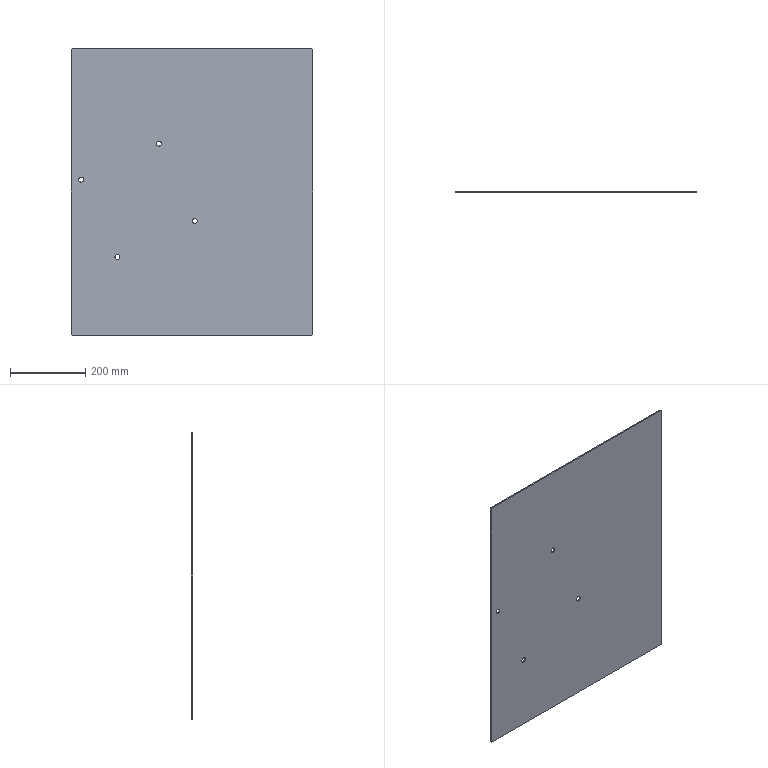Component | SolidWorks | 01-01Chassis-1_01-01-04ChassisWeldment4-1 | 1 solid | 18 faces | box 640 x 3 x 760 mm | volume 1457418 mm3 | cylinder 12 | plane 6 | commonest cylinder face diameters 13.5 x8 10 x4 | material Q235
STEP:
#1=CARTESIAN_POINT('',(-3.474,1.575,4.786));
#2=VERTEX_POINT('',#1);
#3=CARTESIAN_POINT('',(-3.474,1.575,5.317));
#4=VERTEX_POINT('',#3);
#5=CARTESIAN_POINT('',(-3.474,1.575,5.052));
#6=DIRECTION('',(0.,1.,0.));
#7=DIRECTION('',(0.,0.,1.));
#8=AXIS2_PLACEMENT_3D('',#5,#6,#7);
#9=CIRCLE('',#8,0.2657);
#10=EDGE_CURVE('',#2,#4,#9,.T.);
#11=ORIENTED_EDGE('',*,*,#10,.F.);
#12=CARTESIAN_POINT('',(-3.474,1.693,4.786));
#13=VERTEX_POINT('',#12);
#14=CARTESIAN_POINT('',(-3.474,1.575,4.786));
#15=DIRECTION('',(0.,1.,0.));
#16=VECTOR('',#15,39.37);
#17=LINE('',#14,#16);
#18=EDGE_CURVE('',#2,#13,#17,.T.);
#19=ORIENTED_EDGE('',*,*,#18,.T.);
#20=CARTESIAN_POINT('',(-3.474,1.693,5.317));
#21=VERTEX_POINT('',#20);
#22=CARTESIAN_POINT('',(-3.474,1.693,5.052));
#23=DIRECTION('',(0.,1.,0.));
#24=DIRECTION('',(0.,0.,1.));
#25=AXIS2_PLACEMENT_3D('',#22,#23,#24);
#26=CIRCLE('',#25,0.2657);
#27=EDGE_CURVE('',#13,#21,#26,.T.);
#28=ORIENTED_EDGE('',*,*,#27,.T.);
#29=CARTESIAN_POINT('',(-3.474,1.575,5.317));
#30=DIRECTION('',(0.,1.,0.));
#31=VECTOR('',#30,39.37);
#32=LINE('',#29,#31);
#33=EDGE_CURVE('',#4,#21,#32,.T.);
#34=ORIENTED_EDGE('',*,*,#33,.F.);
#35=EDGE_LOOP('',(#11,#19,#28,#34));
#36=FACE_OUTER_BOUND('',#35,.T.);
#37=CARTESIAN_POINT('',(-3.474,1.575,5.052));
#38=DIRECTION('',(0.,1.,0.));
#39=DIRECTION('',(0.,0.,1.));
#40=AXIS2_PLACEMENT_3D('',#37,#38,#39);
#41=CYLINDRICAL_SURFACE('',#40,0.2657);
#42=ADVANCED_FACE('',(#36),#41,.F.);
#43=CARTESIAN_POINT('',(0.291,1.575,-3.288));
#44=VERTEX_POINT('',#43);
#45=CARTESIAN_POINT('',(0.291,1.575,-2.756));
#46=VERTEX_POINT('',#45);
#47=CARTESIAN_POINT('',(0.291,1.575,-3.022));
#48=DIRECTION('',(0.,1.,0.));
#49=DIRECTION('',(0.,0.,1.));
#50=AXIS2_PLACEMENT_3D('',#47,#48,#49);
#51=CIRCLE('',#50,0.2657);
#52=EDGE_CURVE('',#44,#46,#51,.T.);
#53=ORIENTED_EDGE('',*,*,#52,.F.);
#54=CARTESIAN_POINT('',(0.291,1.693,-3.288));
#55=VERTEX_POINT('',#54);
#56=CARTESIAN_POINT('',(0.291,1.575,-3.288));
#57=DIRECTION('',(0.,1.,0.));
#58=VECTOR('',#57,39.37);
#59=LINE('',#56,#58);
#60=EDGE_CURVE('',#44,#55,#59,.T.);
#61=ORIENTED_EDGE('',*,*,#60,.T.);
#62=CARTESIAN_POINT('',(0.291,1.693,-2.756));
#63=VERTEX_POINT('',#62);
#64=CARTESIAN_POINT('',(0.291,1.693,-3.022));
#65=DIRECTION('',(0.,1.,0.));
#66=DIRECTION('',(0.,0.,1.));
#67=AXIS2_PLACEMENT_3D('',#64,#65,#66);
#68=CIRCLE('',#67,0.2657);
#69=EDGE_CURVE('',#55,#63,#68,.T.);
#70=ORIENTED_EDGE('',*,*,#69,.T.);
#71=CARTESIAN_POINT('',(0.291,1.575,-2.756));
#72=DIRECTION('',(0.,1.,0.));
#73=VECTOR('',#72,39.37);
#74=LINE('',#71,#73);
#75=EDGE_CURVE('',#46,#63,#74,.T.);
#76=ORIENTED_EDGE('',*,*,#75,.F.);
#77=EDGE_LOOP('',(#53,#61,#70,#76));
#78=FACE_OUTER_BOUND('',#77,.T.);
#79=CARTESIAN_POINT('',(0.291,1.575,-3.022));
#80=DIRECTION('',(0.,1.,0.));
#81=DIRECTION('',(0.,0.,1.));
#82=AXIS2_PLACEMENT_3D('',#79,#80,#81);
#83=CYLINDRICAL_SURFACE('',#82,0.2657);
#84=ADVANCED_FACE('',(#78),#83,.F.);
#85=CARTESIAN_POINT('',(-7.783,1.575,-7.053));
#86=VERTEX_POINT('',#85);
#87=CARTESIAN_POINT('',(-7.783,1.575,-6.521));
#88=VERTEX_POINT('',#87);
#89=CARTESIAN_POINT('',(-7.783,1.575,-6.787));
#90=DIRECTION('',(0.,1.,0.));
#91=DIRECTION('',(0.,0.,1.));
#92=AXIS2_PLACEMENT_3D('',#89,#90,#91);
#93=CIRCLE('',#92,0.2657);
#94=EDGE_CURVE('',#86,#88,#93,.T.);
#95=ORIENTED_EDGE('',*,*,#94,.F.);
#96=CARTESIAN_POINT('',(-7.783,1.693,-7.053));
#97=VERTEX_POINT('',#96);
#98=CARTESIAN_POINT('',(-7.783,1.575,-7.053));
#99=DIRECTION('',(0.,1.,0.));
#100=VECTOR('',#99,39.37);
#101=LINE('',#98,#100);
#102=EDGE_CURVE('',#86,#97,#101,.T.);
#103=ORIENTED_EDGE('',*,*,#102,.T.);
#104=CARTESIAN_POINT('',(-7.783,1.693,-6.521));
#105=VERTEX_POINT('',#104);
#106=CARTESIAN_POINT('',(-7.783,1.693,-6.787));
#107=DIRECTION('',(0.,1.,0.));
#108=DIRECTION('',(0.,0.,1.));
#109=AXIS2_PLACEMENT_3D('',#106,#107,#108);
#110=CIRCLE('',#109,0.2657);
#111=EDGE_CURVE('',#97,#105,#110,.T.);
#112=ORIENTED_EDGE('',*,*,#111,.T.);
#113=CARTESIAN_POINT('',(-7.783,1.575,-6.521));
#114=DIRECTION('',(0.,1.,0.));
#115=VECTOR('',#114,39.37);
#116=LINE('',#113,#115);
#117=EDGE_CURVE('',#88,#105,#116,.T.);
#118=ORIENTED_EDGE('',*,*,#117,.F.);
#119=EDGE_LOOP('',(#95,#103,#112,#118));
#120=FACE_OUTER_BOUND('',#119,.T.);
#121=CARTESIAN_POINT('',(-7.783,1.575,-6.787));
#122=DIRECTION('',(0.,1.,0.));
#123=DIRECTION('',(0.,0.,1.));
#124=AXIS2_PLACEMENT_3D('',#121,#122,#123);
#125=CYLINDRICAL_SURFACE('',#124,0.2657);
#126=ADVANCED_FACE('',(#120),#125,.F.);
#127=CARTESIAN_POINT('',(-11.548,1.575,1.021));
#128=VERTEX_POINT('',#127);
#129=CARTESIAN_POINT('',(-11.548,1.575,1.553));
#130=VERTEX_POINT('',#129);
#131=CARTESIAN_POINT('',(-11.548,1.575,1.287));
#132=DIRECTION('',(0.,1.,0.));
#133=DIRECTION('',(0.,0.,1.));
#134=AXIS2_PLACEMENT_3D('',#131,#132,#133);
#135=CIRCLE('',#134,0.2657);
#136=EDGE_CURVE('',#128,#130,#135,.T.);
#137=ORIENTED_EDGE('',*,*,#136,.F.);
#138=CARTESIAN_POINT('',(-11.548,1.693,1.021));
#139=VERTEX_POINT('',#138);
#140=CARTESIAN_POINT('',(-11.548,1.575,1.021));
#141=DIRECTION('',(0.,1.,0.));
#142=VECTOR('',#141,39.37);
#143=LINE('',#140,#142);
#144=EDGE_CURVE('',#128,#139,#143,.T.);
#145=ORIENTED_EDGE('',*,*,#144,.T.);
#146=CARTESIAN_POINT('',(-11.548,1.693,1.553));
#147=VERTEX_POINT('',#146);
#148=CARTESIAN_POINT('',(-11.548,1.693,1.287));
#149=DIRECTION('',(0.,1.,0.));
#150=DIRECTION('',(0.,0.,1.));
#151=AXIS2_PLACEMENT_3D('',#148,#149,#150);
#152=CIRCLE('',#151,0.2657);
#153=EDGE_CURVE('',#139,#147,#152,.T.);
#154=ORIENTED_EDGE('',*,*,#153,.T.);
#155=CARTESIAN_POINT('',(-11.548,1.575,1.553));
#156=DIRECTION('',(0.,1.,0.));
#157=VECTOR('',#156,39.37);
#158=LINE('',#155,#157);
#159=EDGE_CURVE('',#130,#147,#158,.T.);
#160=ORIENTED_EDGE('',*,*,#159,.F.);
#161=EDGE_LOOP('',(#137,#145,#154,#160));
#162=FACE_OUTER_BOUND('',#161,.T.);
#163=CARTESIAN_POINT('',(-11.548,1.575,1.287));
#164=DIRECTION('',(0.,1.,0.));
#165=DIRECTION('',(0.,0.,1.));
#166=AXIS2_PLACEMENT_3D('',#163,#164,#165);
#167=CYLINDRICAL_SURFACE('',#166,0.2657);
#168=ADVANCED_FACE('',(#162),#167,.F.);
#169=CARTESIAN_POINT('',(-12.598,1.693,14.764));
#170=VERTEX_POINT('',#169);
#171=CARTESIAN_POINT('',(-12.402,1.693,14.961));
#172=VERTEX_POINT('',#171);
#173=CARTESIAN_POINT('',(-12.402,1.693,14.764));
#174=DIRECTION('',(0.,1.,0.));
#175=DIRECTION('',(0.,0.,-1.));
#176=AXIS2_PLACEMENT_3D('',#173,#174,#175);
#177=CIRCLE('',#176,0.1969);
#178=EDGE_CURVE('',#170,#172,#177,.T.);
#179=ORIENTED_EDGE('',*,*,#178,.F.);
#180=CARTESIAN_POINT('',(-12.598,1.575,14.764));
#181=VERTEX_POINT('',#180);
#182=CARTESIAN_POINT('',(-12.598,1.575,14.764));
#183=DIRECTION('',(0.,1.,0.));
#184=VECTOR('',#183,39.37);
#185=LINE('',#182,#184);
#186=EDGE_CURVE('',#181,#170,#185,.T.);
#187=ORIENTED_EDGE('',*,*,#186,.F.);
#188=CARTESIAN_POINT('',(-12.402,1.575,14.961));
#189=VERTEX_POINT('',#188);
#190=CARTESIAN_POINT('',(-12.402,1.575,14.764));
#191=DIRECTION('',(0.,1.,0.));
#192=DIRECTION('',(0.,0.,-1.));
#193=AXIS2_PLACEMENT_3D('',#190,#191,#192);
#194=CIRCLE('',#193,0.1969);
#195=EDGE_CURVE('',#181,#189,#194,.T.);
#196=ORIENTED_EDGE('',*,*,#195,.T.);
#197=CARTESIAN_POINT('',(-12.402,1.575,14.961));
#198=DIRECTION('',(0.,1.,0.));
#199=VECTOR('',#198,39.37);
#200=LINE('',#197,#199);
#201=EDGE_CURVE('',#189,#172,#200,.T.);
#202=ORIENTED_EDGE('',*,*,#201,.T.);
#203=EDGE_LOOP('',(#179,#187,#196,#202));
#204=FACE_OUTER_BOUND('',#203,.T.);
#205=CARTESIAN_POINT('',(-12.402,1.575,14.764));
#206=DIRECTION('',(0.,1.,0.));
#207=DIRECTION('',(0.,0.,1.));
#208=AXIS2_PLACEMENT_3D('',#205,#206,#207);
#209=CYLINDRICAL_SURFACE('',#208,0.1969);
#210=ADVANCED_FACE('',(#204),#209,.T.);
#211=CARTESIAN_POINT('',(-12.598,1.693,-14.764));
#212=VERTEX_POINT('',#211);
#213=CARTESIAN_POINT('',(-12.598,1.693,14.764));
#214=DIRECTION('',(0.,0.,1.));
#215=VECTOR('',#214,39.37);
#216=LINE('',#213,#215);
#217=EDGE_CURVE('',#212,#170,#216,.T.);
#218=ORIENTED_EDGE('',*,*,#217,.F.);
#219=CARTESIAN_POINT('',(-12.598,1.575,-14.764));
#220=VERTEX_POINT('',#219);
#221=CARTESIAN_POINT('',(-12.598,1.575,-14.764));
#222=DIRECTION('',(0.,1.,0.));
#223=VECTOR('',#222,39.37);
#224=LINE('',#221,#223);
#225=EDGE_CURVE('',#220,#212,#224,.T.);
#226=ORIENTED_EDGE('',*,*,#225,.F.);
#227=CARTESIAN_POINT('',(-12.598,1.575,14.764));
#228=DIRECTION('',(0.,0.,1.));
#229=VECTOR('',#228,39.37);
#230=LINE('',#227,#229);
#231=EDGE_CURVE('',#220,#181,#230,.T.);
#232=ORIENTED_EDGE('',*,*,#231,.T.);
#233=ORIENTED_EDGE('',*,*,#186,.T.);
#234=EDGE_LOOP('',(#218,#226,#232,#233));
#235=FACE_OUTER_BOUND('',#234,.T.);
#236=CARTESIAN_POINT('',(-12.598,1.575,14.764));
#237=DIRECTION('',(-1.,0.,0.));
#238=DIRECTION('',(0.,0.,1.));
#239=AXIS2_PLACEMENT_3D('',#236,#237,#238);
#240=PLANE('',#239);
#241=ADVANCED_FACE('',(#235),#240,.T.);
#242=CARTESIAN_POINT('',(-12.402,1.693,-14.961));
#243=VERTEX_POINT('',#242);
#244=CARTESIAN_POINT('',(-12.402,1.693,-14.764));
#245=DIRECTION('',(0.,1.,0.));
#246=DIRECTION('',(0.,0.,1.));
#247=AXIS2_PLACEMENT_3D('',#244,#245,#246);
#248=CIRCLE('',#247,0.1969);
#249=EDGE_CURVE('',#243,#212,#248,.T.);
#250=ORIENTED_EDGE('',*,*,#249,.F.);
#251=CARTESIAN_POINT('',(-12.402,1.575,-14.961));
#252=VERTEX_POINT('',#251);
#253=CARTESIAN_POINT('',(-12.402,1.575,-14.961));
#254=DIRECTION('',(0.,1.,0.));
#255=VECTOR('',#254,39.37);
#256=LINE('',#253,#255);
#257=EDGE_CURVE('',#252,#243,#256,.T.);
#258=ORIENTED_EDGE('',*,*,#257,.F.);
#259=CARTESIAN_POINT('',(-12.402,1.575,-14.764));
#260=DIRECTION('',(0.,1.,0.));
#261=DIRECTION('',(0.,0.,1.));
#262=AXIS2_PLACEMENT_3D('',#259,#260,#261);
#263=CIRCLE('',#262,0.1969);
#264=EDGE_CURVE('',#252,#220,#263,.T.);
#265=ORIENTED_EDGE('',*,*,#264,.T.);
#266=ORIENTED_EDGE('',*,*,#225,.T.);
#267=EDGE_LOOP('',(#250,#258,#265,#266));
#268=FACE_OUTER_BOUND('',#267,.T.);
#269=CARTESIAN_POINT('',(-12.402,1.575,-14.764));
#270=DIRECTION('',(0.,1.,0.));
#271=DIRECTION('',(0.,0.,1.));
#272=AXIS2_PLACEMENT_3D('',#269,#270,#271);
#273=CYLINDRICAL_SURFACE('',#272,0.1969);
#274=ADVANCED_FACE('',(#268),#273,.T.);
#275=CARTESIAN_POINT('',(12.402,1.693,-14.961));
#276=VERTEX_POINT('',#275);
#277=CARTESIAN_POINT('',(12.402,1.693,-14.961));
#278=DIRECTION('',(-1.,0.,0.));
#279=VECTOR('',#278,39.37);
#280=LINE('',#277,#279);
#281=EDGE_CURVE('',#276,#243,#280,.T.);
#282=ORIENTED_EDGE('',*,*,#281,.F.);
#283=CARTESIAN_POINT('',(12.402,1.575,-14.961));
#284=VERTEX_POINT('',#283);
#285=CARTESIAN_POINT('',(12.402,1.575,-14.961));
#286=DIRECTION('',(0.,1.,0.));
#287=VECTOR('',#286,39.37);
#288=LINE('',#285,#287);
#289=EDGE_CURVE('',#284,#276,#288,.T.);
#290=ORIENTED_EDGE('',*,*,#289,.F.);
#291=CARTESIAN_POINT('',(12.402,1.575,-14.961));
#292=DIRECTION('',(-1.,0.,0.));
#293=VECTOR('',#292,39.37);
#294=LINE('',#291,#293);
#295=EDGE_CURVE('',#284,#252,#294,.T.);
#296=ORIENTED_EDGE('',*,*,#295,.T.);
#297=ORIENTED_EDGE('',*,*,#257,.T.);
#298=EDGE_LOOP('',(#282,#290,#296,#297));
#299=FACE_OUTER_BOUND('',#298,.T.);
#300=CARTESIAN_POINT('',(12.402,1.575,-14.961));
#301=DIRECTION('',(-0.,0.,-1.));
#302=DIRECTION('',(-1.,0.,0.));
#303=AXIS2_PLACEMENT_3D('',#300,#301,#302);
#304=PLANE('',#303);
#305=ADVANCED_FACE('',(#299),#304,.T.);
#306=CARTESIAN_POINT('',(12.598,1.693,-14.764));
#307=VERTEX_POINT('',#306);
#308=CARTESIAN_POINT('',(12.402,1.693,-14.764));
#309=DIRECTION('',(0.,1.,0.));
#310=DIRECTION('',(0.,0.,1.));
#311=AXIS2_PLACEMENT_3D('',#308,#309,#310);
#312=CIRCLE('',#311,0.1969);
#313=EDGE_CURVE('',#307,#276,#312,.T.);
#314=ORIENTED_EDGE('',*,*,#313,.F.);
#315=CARTESIAN_POINT('',(12.598,1.575,-14.764));
#316=VERTEX_POINT('',#315);
#317=CARTESIAN_POINT('',(12.598,1.575,-14.764));
#318=DIRECTION('',(0.,1.,0.));
#319=VECTOR('',#318,39.37);
#320=LINE('',#317,#319);
#321=EDGE_CURVE('',#316,#307,#320,.T.);
#322=ORIENTED_EDGE('',*,*,#321,.F.);
#323=CARTESIAN_POINT('',(12.402,1.575,-14.764));
#324=DIRECTION('',(0.,1.,0.));
#325=DIRECTION('',(0.,0.,1.));
#326=AXIS2_PLACEMENT_3D('',#323,#324,#325);
#327=CIRCLE('',#326,0.1969);
#328=EDGE_CURVE('',#316,#284,#327,.T.);
#329=ORIENTED_EDGE('',*,*,#328,.T.);
#330=ORIENTED_EDGE('',*,*,#289,.T.);
#331=EDGE_LOOP('',(#314,#322,#329,#330));
#332=FACE_OUTER_BOUND('',#331,.T.);
#333=CARTESIAN_POINT('',(12.402,1.575,-14.764));
#334=DIRECTION('',(0.,1.,0.));
#335=DIRECTION('',(0.,0.,1.));
#336=AXIS2_PLACEMENT_3D('',#333,#334,#335);
#337=CYLINDRICAL_SURFACE('',#336,0.1969);
#338=ADVANCED_FACE('',(#332),#337,.T.);
#339=CARTESIAN_POINT('',(12.598,1.693,14.764));
#340=VERTEX_POINT('',#339);
#341=CARTESIAN_POINT('',(12.598,1.693,14.764));
#342=DIRECTION('',(0.,0.,-1.));
#343=VECTOR('',#342,39.37);
#344=LINE('',#341,#343);
#345=EDGE_CURVE('',#340,#307,#344,.T.);
#346=ORIENTED_EDGE('',*,*,#345,.F.);
#347=CARTESIAN_POINT('',(12.598,1.575,14.764));
#348=VERTEX_POINT('',#347);
#349=CARTESIAN_POINT('',(12.598,1.575,14.764));
#350=DIRECTION('',(0.,1.,0.));
#351=VECTOR('',#350,39.37);
#352=LINE('',#349,#351);
#353=EDGE_CURVE('',#348,#340,#352,.T.);
#354=ORIENTED_EDGE('',*,*,#353,.F.);
#355=CARTESIAN_POINT('',(12.598,1.575,14.764));
#356=DIRECTION('',(0.,0.,-1.));
#357=VECTOR('',#356,39.37);
#358=LINE('',#355,#357);
#359=EDGE_CURVE('',#348,#316,#358,.T.);
#360=ORIENTED_EDGE('',*,*,#359,.T.);
#361=ORIENTED_EDGE('',*,*,#321,.T.);
#362=EDGE_LOOP('',(#346,#354,#360,#361));
#363=FACE_OUTER_BOUND('',#362,.T.);
#364=CARTESIAN_POINT('',(12.598,1.575,14.764));
#365=DIRECTION('',(1.,0.,0.));
#366=DIRECTION('',(0.,0.,-1.));
#367=AXIS2_PLACEMENT_3D('',#364,#365,#366);
#368=PLANE('',#367);
#369=ADVANCED_FACE('',(#363),#368,.T.);
#370=CARTESIAN_POINT('',(12.402,1.693,14.961));
#371=VERTEX_POINT('',#370);
#372=CARTESIAN_POINT('',(12.402,1.693,14.764));
#373=DIRECTION('',(0.,1.,0.));
#374=DIRECTION('',(0.,0.,1.));
#375=AXIS2_PLACEMENT_3D('',#372,#373,#374);
#376=CIRCLE('',#375,0.1969);
#377=EDGE_CURVE('',#371,#340,#376,.T.);
#378=ORIENTED_EDGE('',*,*,#377,.F.);
#379=CARTESIAN_POINT('',(12.402,1.575,14.961));
#380=VERTEX_POINT('',#379);
#381=CARTESIAN_POINT('',(12.402,1.575,14.961));
#382=DIRECTION('',(0.,1.,0.));
#383=VECTOR('',#382,39.37);
#384=LINE('',#381,#383);
#385=EDGE_CURVE('',#380,#371,#384,.T.);
#386=ORIENTED_EDGE('',*,*,#385,.F.);
#387=CARTESIAN_POINT('',(12.402,1.575,14.764));
#388=DIRECTION('',(0.,1.,0.));
#389=DIRECTION('',(0.,0.,1.));
#390=AXIS2_PLACEMENT_3D('',#387,#388,#389);
#391=CIRCLE('',#390,0.1969);
#392=EDGE_CURVE('',#380,#348,#391,.T.);
#393=ORIENTED_EDGE('',*,*,#392,.T.);
#394=ORIENTED_EDGE('',*,*,#353,.T.);
#395=EDGE_LOOP('',(#378,#386,#393,#394));
#396=FACE_OUTER_BOUND('',#395,.T.);
#397=CARTESIAN_POINT('',(12.402,1.575,14.764));
#398=DIRECTION('',(0.,1.,0.));
#399=DIRECTION('',(0.,0.,1.));
#400=AXIS2_PLACEMENT_3D('',#397,#398,#399);
#401=CYLINDRICAL_SURFACE('',#400,0.1969);
#402=ADVANCED_FACE('',(#396),#401,.T.);
#403=CARTESIAN_POINT('',(12.402,1.693,14.961));
#404=DIRECTION('',(1.,0.,-0.));
#405=VECTOR('',#404,39.37);
#406=LINE('',#403,#405);
#407=EDGE_CURVE('',#172,#371,#406,.T.);
#408=ORIENTED_EDGE('',*,*,#407,.F.);
#409=ORIENTED_EDGE('',*,*,#201,.F.);
#410=CARTESIAN_POINT('',(12.402,1.575,14.961));
#411=DIRECTION('',(1.,0.,-0.));
#412=VECTOR('',#411,39.37);
#413=LINE('',#410,#412);
#414=EDGE_CURVE('',#189,#380,#413,.T.);
#415=ORIENTED_EDGE('',*,*,#414,.T.);
#416=ORIENTED_EDGE('',*,*,#385,.T.);
#417=EDGE_LOOP('',(#408,#409,#415,#416));
#418=FACE_OUTER_BOUND('',#417,.T.);
#419=CARTESIAN_POINT('',(12.402,1.575,14.961));
#420=DIRECTION('',(0.,0.,1.));
#421=DIRECTION('',(1.,0.,-0.));
#422=AXIS2_PLACEMENT_3D('',#419,#420,#421);
#423=PLANE('',#422);
#424=ADVANCED_FACE('',(#418),#423,.T.);
#425=CARTESIAN_POINT('',(-3.474,1.575,5.052));
#426=DIRECTION('',(0.,1.,0.));
#427=DIRECTION('',(0.,0.,1.));
#428=AXIS2_PLACEMENT_3D('',#425,#426,#427);
#429=CIRCLE('',#428,0.2657);
#430=EDGE_CURVE('',#4,#2,#429,.T.);
#431=ORIENTED_EDGE('',*,*,#430,.T.);
#432=ORIENTED_EDGE('',*,*,#10,.T.);
#433=EDGE_LOOP('',(#431,#432));
#434=FACE_BOUND('',#433,.T.);
#435=CARTESIAN_POINT('',(0.291,1.575,-3.022));
#436=DIRECTION('',(0.,1.,0.));
#437=DIRECTION('',(0.,0.,1.));
#438=AXIS2_PLACEMENT_3D('',#435,#436,#437);
#439=CIRCLE('',#438,0.2657);
#440=EDGE_CURVE('',#46,#44,#439,.T.);
#441=ORIENTED_EDGE('',*,*,#440,.T.);
#442=ORIENTED_EDGE('',*,*,#52,.T.);
#443=EDGE_LOOP('',(#441,#442));
#444=FACE_BOUND('',#443,.T.);
#445=CARTESIAN_POINT('',(-7.783,1.575,-6.787));
#446=DIRECTION('',(0.,1.,0.));
#447=DIRECTION('',(0.,0.,1.));
#448=AXIS2_PLACEMENT_3D('',#445,#446,#447);
#449=CIRCLE('',#448,0.2657);
#450=EDGE_CURVE('',#88,#86,#449,.T.);
#451=ORIENTED_EDGE('',*,*,#450,.T.);
#452=ORIENTED_EDGE('',*,*,#94,.T.);
#453=EDGE_LOOP('',(#451,#452));
#454=FACE_BOUND('',#453,.T.);
#455=CARTESIAN_POINT('',(-11.548,1.575,1.287));
#456=DIRECTION('',(0.,1.,0.));
#457=DIRECTION('',(0.,0.,1.));
#458=AXIS2_PLACEMENT_3D('',#455,#456,#457);
#459=CIRCLE('',#458,0.2657);
#460=EDGE_CURVE('',#130,#128,#459,.T.);
#461=ORIENTED_EDGE('',*,*,#460,.T.);
#462=ORIENTED_EDGE('',*,*,#136,.T.);
#463=EDGE_LOOP('',(#461,#462));
#464=FACE_BOUND('',#463,.T.);
#465=ORIENTED_EDGE('',*,*,#195,.F.);
#466=ORIENTED_EDGE('',*,*,#231,.F.);
#467=ORIENTED_EDGE('',*,*,#264,.F.);
#468=ORIENTED_EDGE('',*,*,#295,.F.);
#469=ORIENTED_EDGE('',*,*,#328,.F.);
#470=ORIENTED_EDGE('',*,*,#359,.F.);
#471=ORIENTED_EDGE('',*,*,#392,.F.);
#472=ORIENTED_EDGE('',*,*,#414,.F.);
#473=EDGE_LOOP('',(#465,#466,#467,#468,#469,#470,#471,#472));
#474=FACE_OUTER_BOUND('',#473,.T.);
#475=CARTESIAN_POINT('',(-12.402,1.575,14.764));
#476=DIRECTION('',(0.,-1.,0.));
#477=DIRECTION('',(0.,0.,-1.));
#478=AXIS2_PLACEMENT_3D('',#475,#476,#477);
#479=PLANE('',#478);
#480=ADVANCED_FACE('',(#434,#444,#454,#464,#474),#479,.T.);
#481=CARTESIAN_POINT('',(-3.474,1.693,5.052));
#482=DIRECTION('',(0.,1.,0.));
#483=DIRECTION('',(0.,0.,1.));
#484=AXIS2_PLACEMENT_3D('',#481,#482,#483);
#485=CIRCLE('',#484,0.2657);
#486=EDGE_CURVE('',#21,#13,#485,.T.);
#487=ORIENTED_EDGE('',*,*,#486,.F.);
#488=ORIENTED_EDGE('',*,*,#27,.F.);
#489=EDGE_LOOP('',(#487,#488));
#490=FACE_BOUND('',#489,.T.);
#491=CARTESIAN_POINT('',(0.291,1.693,-3.022));
#492=DIRECTION('',(0.,1.,0.));
#493=DIRECTION('',(0.,0.,1.));
#494=AXIS2_PLACEMENT_3D('',#491,#492,#493);
#495=CIRCLE('',#494,0.2657);
#496=EDGE_CURVE('',#63,#55,#495,.T.);
#497=ORIENTED_EDGE('',*,*,#496,.F.);
#498=ORIENTED_EDGE('',*,*,#69,.F.);
#499=EDGE_LOOP('',(#497,#498));
#500=FACE_BOUND('',#499,.T.);
#501=CARTESIAN_POINT('',(-7.783,1.693,-6.787));
#502=DIRECTION('',(0.,1.,0.));
#503=DIRECTION('',(0.,0.,1.));
#504=AXIS2_PLACEMENT_3D('',#501,#502,#503);
#505=CIRCLE('',#504,0.2657);
#506=EDGE_CURVE('',#105,#97,#505,.T.);
#507=ORIENTED_EDGE('',*,*,#506,.F.);
#508=ORIENTED_EDGE('',*,*,#111,.F.);
#509=EDGE_LOOP('',(#507,#508));
#510=FACE_BOUND('',#509,.T.);
#511=CARTESIAN_POINT('',(-11.548,1.693,1.287));
#512=DIRECTION('',(0.,1.,0.));
#513=DIRECTION('',(0.,0.,1.));
#514=AXIS2_PLACEMENT_3D('',#511,#512,#513);
#515=CIRCLE('',#514,0.2657);
#516=EDGE_CURVE('',#147,#139,#515,.T.);
#517=ORIENTED_EDGE('',*,*,#516,.F.);
#518=ORIENTED_EDGE('',*,*,#153,.F.);
#519=EDGE_LOOP('',(#517,#518));
#520=FACE_BOUND('',#519,.T.);
#521=ORIENTED_EDGE('',*,*,#178,.T.);
#522=ORIENTED_EDGE('',*,*,#407,.T.);
#523=ORIENTED_EDGE('',*,*,#377,.T.);
#524=ORIENTED_EDGE('',*,*,#345,.T.);
#525=ORIENTED_EDGE('',*,*,#313,.T.);
#526=ORIENTED_EDGE('',*,*,#281,.T.);
#527=ORIENTED_EDGE('',*,*,#249,.T.);
#528=ORIENTED_EDGE('',*,*,#217,.T.);
#529=EDGE_LOOP('',(#521,#522,#523,#524,#525,#526,#527,#528));
#530=FACE_OUTER_BOUND('',#529,.T.);
#531=CARTESIAN_POINT('',(-12.402,1.693,14.764));
#532=DIRECTION('',(0.,-1.,0.));
#533=DIRECTION('',(0.,0.,-1.));
#534=AXIS2_PLACEMENT_3D('',#531,#532,#533);
#535=PLANE('',#534);
#536=ADVANCED_FACE('',(#490,#500,#510,#520,#530),#535,.F.);
#537=ORIENTED_EDGE('',*,*,#144,.F.);
#538=ORIENTED_EDGE('',*,*,#460,.F.);
#539=ORIENTED_EDGE('',*,*,#159,.T.);
#540=ORIENTED_EDGE('',*,*,#516,.T.);
#541=EDGE_LOOP('',(#537,#538,#539,#540));
#542=FACE_OUTER_BOUND('',#541,.T.);
#543=CARTESIAN_POINT('',(-11.548,1.575,1.287));
#544=DIRECTION('',(0.,1.,0.));
#545=DIRECTION('',(0.,0.,1.));
#546=AXIS2_PLACEMENT_3D('',#543,#544,#545);
#547=CYLINDRICAL_SURFACE('',#546,0.2657);
#548=ADVANCED_FACE('',(#542),#547,.F.);
#549=ORIENTED_EDGE('',*,*,#102,.F.);
#550=ORIENTED_EDGE('',*,*,#450,.F.);
#551=ORIENTED_EDGE('',*,*,#117,.T.);
#552=ORIENTED_EDGE('',*,*,#506,.T.);
#553=EDGE_LOOP('',(#549,#550,#551,#552));
#554=FACE_OUTER_BOUND('',#553,.T.);
#555=CARTESIAN_POINT('',(-7.783,1.575,-6.787));
#556=DIRECTION('',(0.,1.,0.));
#557=DIRECTION('',(0.,0.,1.));
#558=AXIS2_PLACEMENT_3D('',#555,#556,#557);
#559=CYLINDRICAL_SURFACE('',#558,0.2657);
#560=ADVANCED_FACE('',(#554),#559,.F.);
#561=ORIENTED_EDGE('',*,*,#60,.F.);
#562=ORIENTED_EDGE('',*,*,#440,.F.);
#563=ORIENTED_EDGE('',*,*,#75,.T.);
#564=ORIENTED_EDGE('',*,*,#496,.T.);
#565=EDGE_LOOP('',(#561,#562,#563,#564));
#566=FACE_OUTER_BOUND('',#565,.T.);
#567=CARTESIAN_POINT('',(0.291,1.575,-3.022));
#568=DIRECTION('',(0.,1.,0.));
#569=DIRECTION('',(0.,0.,1.));
#570=AXIS2_PLACEMENT_3D('',#567,#568,#569);
#571=CYLINDRICAL_SURFACE('',#570,0.2657);
#572=ADVANCED_FACE('',(#566),#571,.F.);
#573=ORIENTED_EDGE('',*,*,#18,.F.);
#574=ORIENTED_EDGE('',*,*,#430,.F.);
#575=ORIENTED_EDGE('',*,*,#33,.T.);
#576=ORIENTED_EDGE('',*,*,#486,.T.);
#577=EDGE_LOOP('',(#573,#574,#575,#576));
#578=FACE_OUTER_BOUND('',#577,.T.);
#579=CARTESIAN_POINT('',(-3.474,1.575,5.052));
#580=DIRECTION('',(0.,1.,0.));
#581=DIRECTION('',(0.,0.,1.));
#582=AXIS2_PLACEMENT_3D('',#579,#580,#581);
#583=CYLINDRICAL_SURFACE('',#582,0.2657);
#584=ADVANCED_FACE('',(#578),#583,.F.);
#585=CLOSED_SHELL('',(#42,#84,#126,#168,#210,#241,#274,#305,#338,#369,#402,#424,#480,#536,#548,#560,#572,#584));
#586=MANIFOLD_SOLID_BREP('',#585);
#587=CARTESIAN_POINT('',(0.,0.,0.));
#588=DIRECTION('',(0.,0.,1.));
#589=DIRECTION('',(1.,0.,0.));
#590=AXIS2_PLACEMENT_3D('',#587,#588,#589);
#591=(LENGTH_UNIT()NAMED_UNIT(*)SI_UNIT($,.METRE.));
#592=LENGTH_MEASURE_WITH_UNIT(LENGTH_MEASURE(0.0254),#591);
#593=DIMENSIONAL_EXPONENTS(1.,0.,0.,0.,0.,0.,0.);
#594=(CONVERSION_BASED_UNIT('',#592)LENGTH_UNIT()NAMED_UNIT(#593));
#595=UNCERTAINTY_MEASURE_WITH_UNIT(LENGTH_MEASURE(0.00001),#594,'','');
#596=(NAMED_UNIT(*)PLANE_ANGLE_UNIT()SI_UNIT($,.RADIAN.));
#597=(NAMED_UNIT(*)SI_UNIT($,.STERADIAN.)SOLID_ANGLE_UNIT());
#598=(GEOMETRIC_REPRESENTATION_CONTEXT(3)GLOBAL_UNCERTAINTY_ASSIGNED_CONTEXT((#595))GLOBAL_UNIT_ASSIGNED_CONTEXT((#594,#596,#597))REPRESENTATION_CONTEXT('',''));
#599=ADVANCED_BREP_SHAPE_REPRESENTATION('',(#586,#590),#598);
#600=COLOUR_RGB('',0.7922,0.8196,0.9333);
#601=FILL_AREA_STYLE_COLOUR('',#600);
#602=FILL_AREA_STYLE('',(#601));
#603=SURFACE_STYLE_FILL_AREA(#602);
#604=SURFACE_SIDE_STYLE('',(#603));
#605=SURFACE_STYLE_USAGE(.BOTH.,#604);
#606=PRESENTATION_STYLE_ASSIGNMENT((#605));
#607=STYLED_ITEM('',(#606),#586);
#608=(LENGTH_UNIT()NAMED_UNIT(*)SI_UNIT($,.METRE.));
#609=LENGTH_MEASURE_WITH_UNIT(LENGTH_MEASURE(0.0254),#608);
#610=DIMENSIONAL_EXPONENTS(1.,0.,0.,0.,0.,0.,0.);
#611=(CONVERSION_BASED_UNIT('',#609)LENGTH_UNIT()NAMED_UNIT(#610));
#612=UNCERTAINTY_MEASURE_WITH_UNIT(LENGTH_MEASURE(0.00001),#611,'','');
#613=(NAMED_UNIT(*)PLANE_ANGLE_UNIT()SI_UNIT($,.RADIAN.));
#614=(NAMED_UNIT(*)SI_UNIT($,.STERADIAN.)SOLID_ANGLE_UNIT());
#615=(GEOMETRIC_REPRESENTATION_CONTEXT(3)GLOBAL_UNCERTAINTY_ASSIGNED_CONTEXT((#612))GLOBAL_UNIT_ASSIGNED_CONTEXT((#611,#613,#614))REPRESENTATION_CONTEXT('',''));
#616=MECHANICAL_DESIGN_GEOMETRIC_PRESENTATION_REPRESENTATION('',(#607),#615);
#617=PRESENTATION_LAYER_ASSIGNMENT('','',(#607));